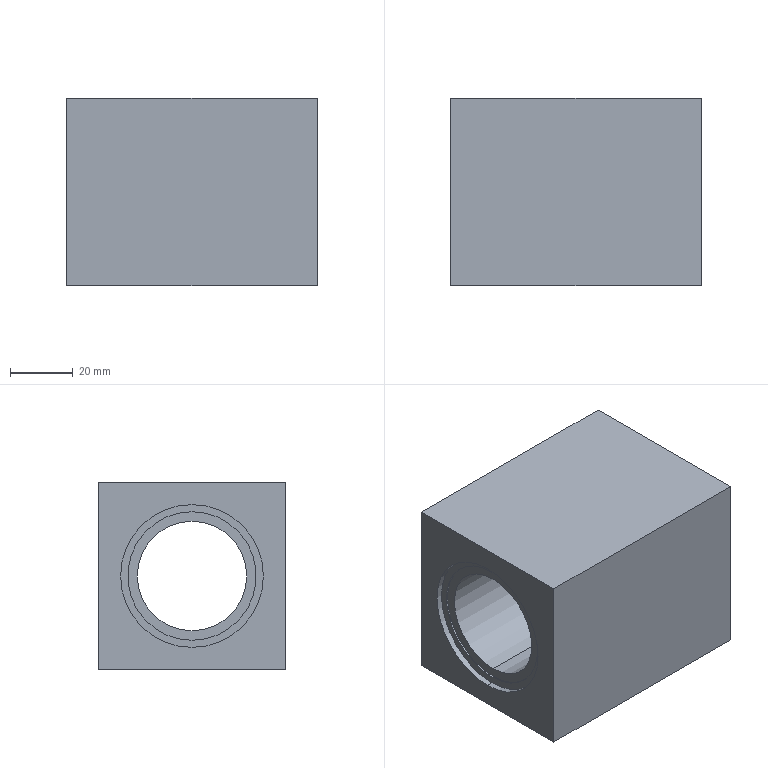Component | SolidWorks | RMS32X800_0-1_RMS32X50_Body-1 | 1 solid | 56 faces | volume 206984 mm3 | cylinder 26 | cone 16 | plane 14 | commonest cylinder face diameters 6 x8 4.5 x8 41.095 x4 45.667 x4 35 x2